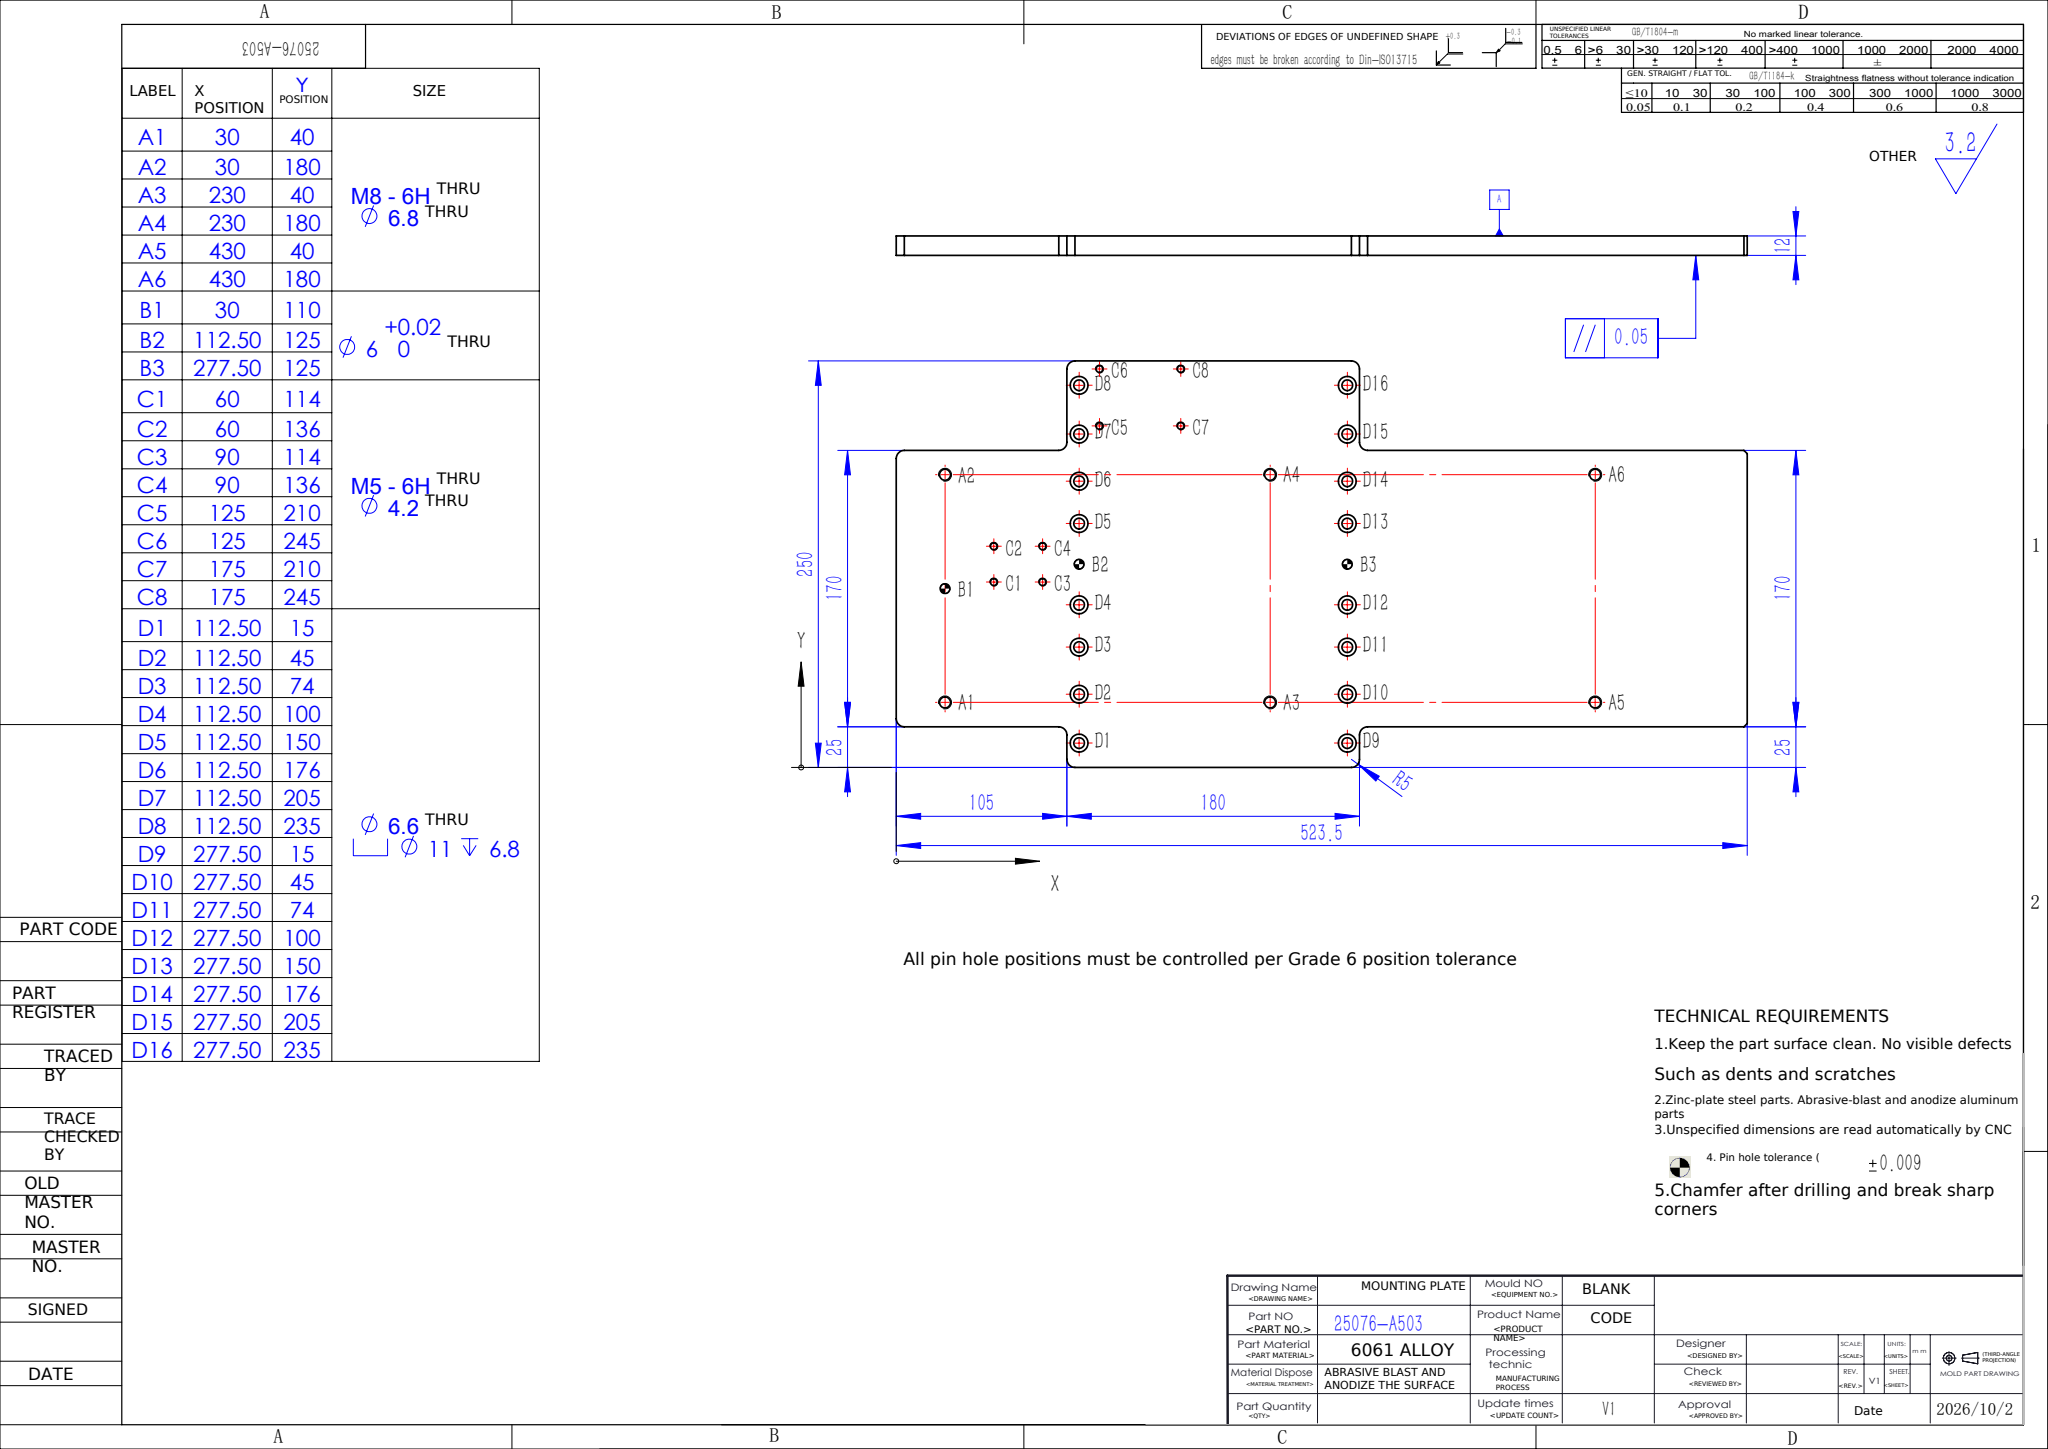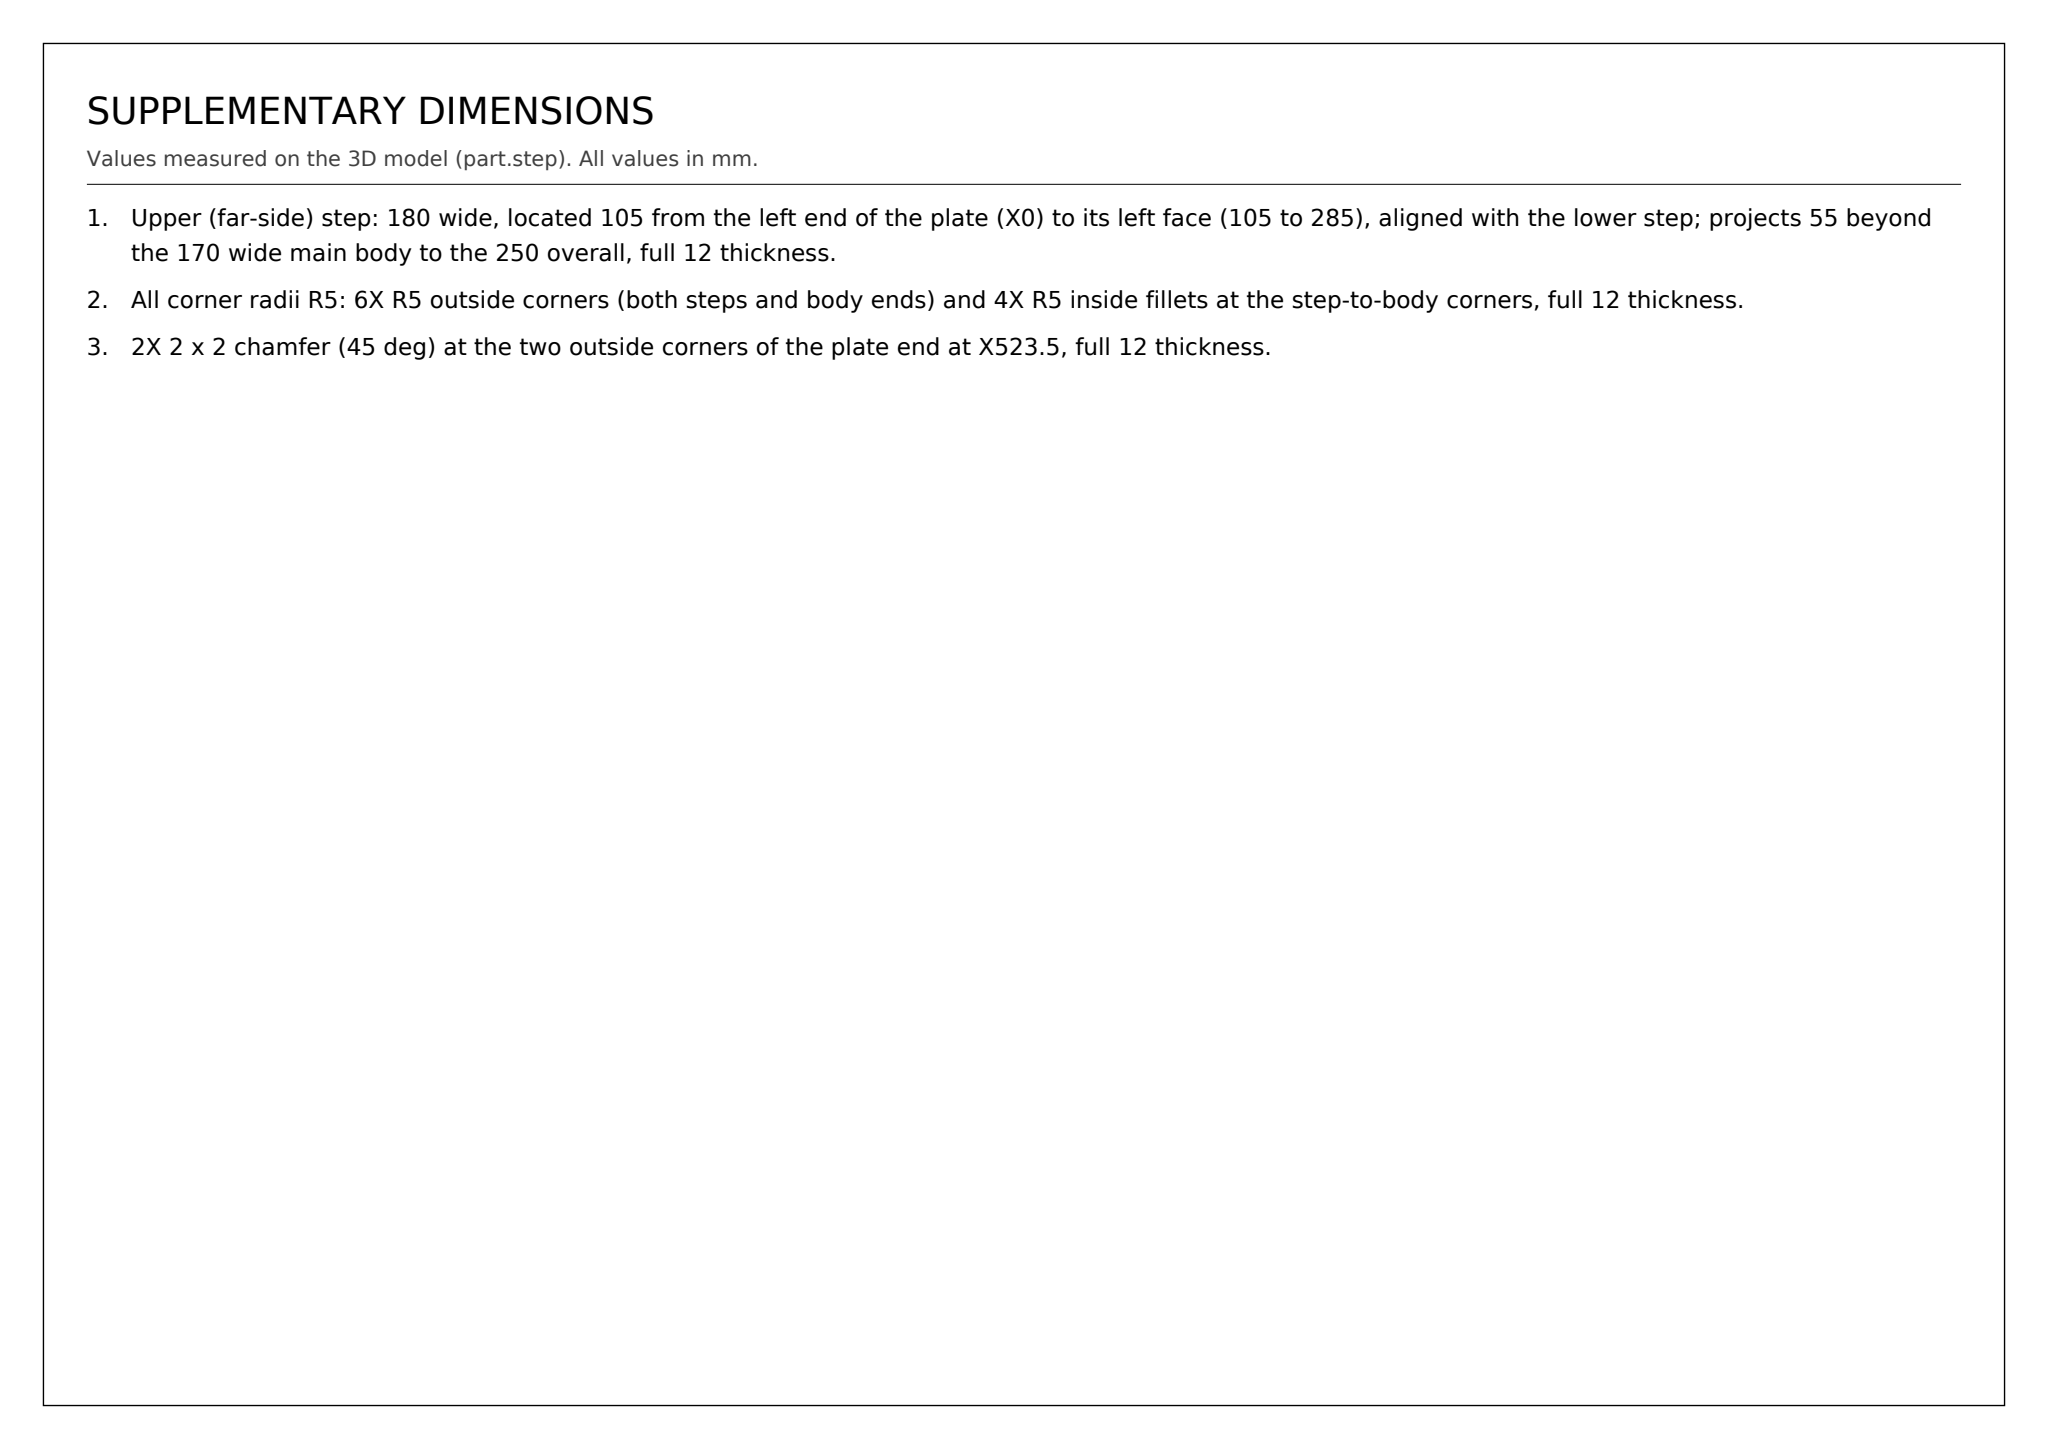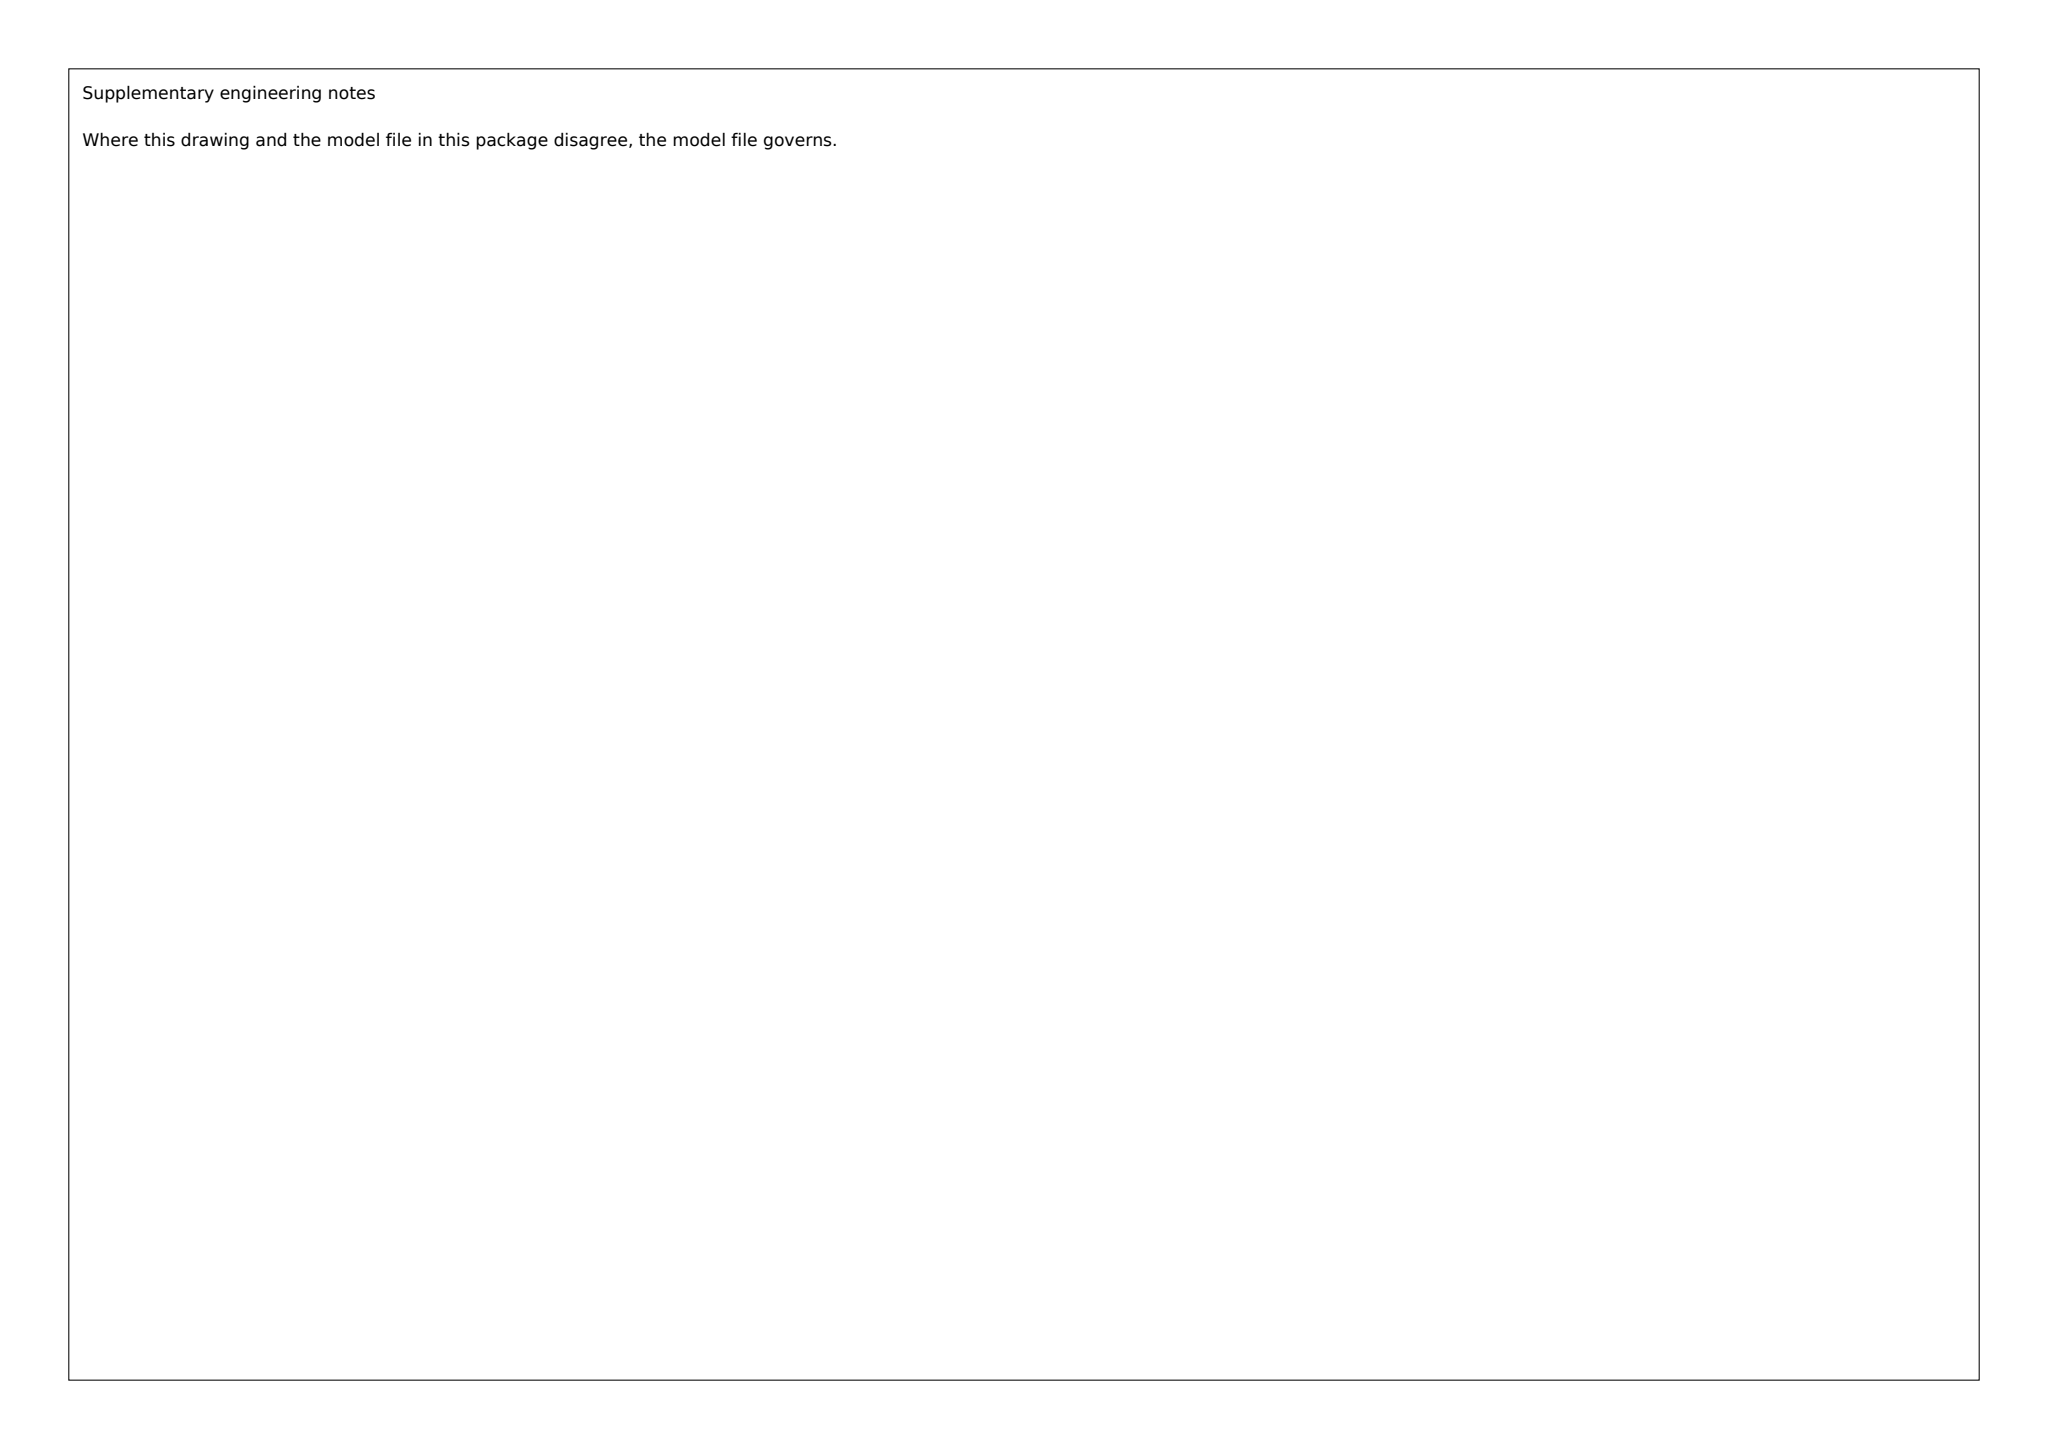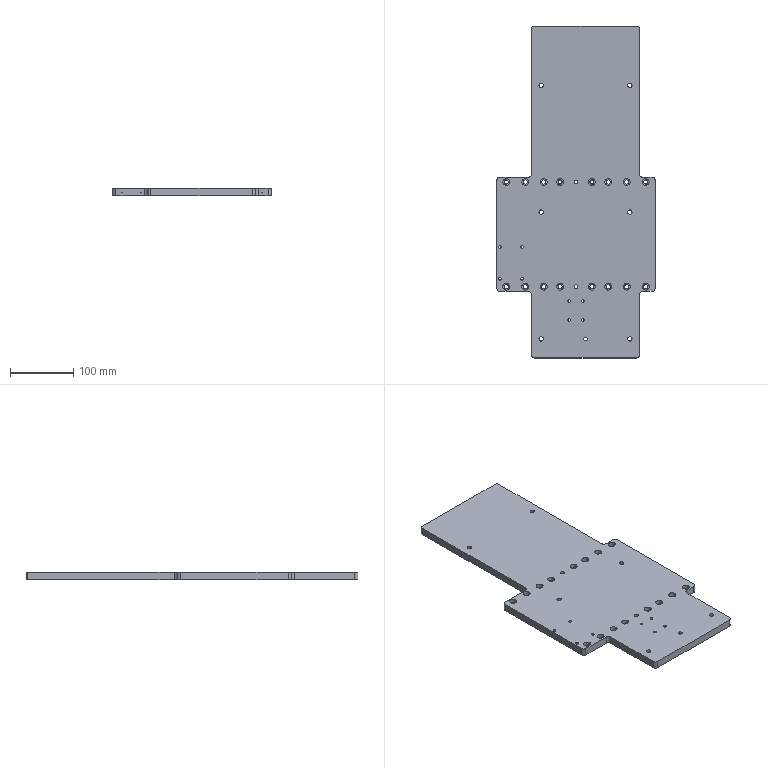Part | SolidWorks | mm | 1 solid | 140 faces | box 250 x 523.5 x 12 mm | volume 1222414 mm3 | cylinder 108 | plane 32 | commonest cylinder face diameters 11 x32 6.6 x32 4.2 x16 6.8 x12 10 x10 6 x6
Drawing notes:
Upper (far-side) step: 180 wide, located 105 from the left end of the plate (X0) to its left face (105 to 285), aligned with the lower step; projects 55 beyond the 170 wide main body to the 250 overall, full 12 thickness. | from the solid: Narrow main body faces at x=55 and x=225 (170 wide) run the full length; the wide section spans x=0 to 250 only between y=105 and y=285 (180 long, i.e. 105 from the y=0 end). Projections are therefore 55 (x 0-55, drawing upper side, since drawing Y = 250 - STEP x per A2 at Y180 = STEP x70) and 25 (x 225-250, drawing lower side); all faces extend z 0 to 12.
All corner radii R5: 6X R5 outside corners (both steps and body ends) and 4X R5 inside fillets at the step-to-body corners, full 12 thickness. | from the solid: cylinders: 6 convex arcs Ø10 (R5) 90 deg z 0-12 at (220,5),(60,5),(245,110),(245,280),(5,110),(5,280) and 4 concave arcs Ø10 (R5) 90 deg z 0-12 at (230,100),(230,290),(50,100),(50,290)
2X 2 x 2 chamfer (45 deg) at the two outside corners of the plate end at X523.5, full 12 thickness. | from the solid: inclined_planes 45/45/90 at bbox_from (223,521.5,0) and (55,521.5,0), size 2 x 2 x 12
build123d program:
from build123d import *

# Parameters (mm, degrees)
SKETCH1_W                                           = 140
SKETCH1_H                                           = 630
BOSS_EXTRUDE1_DEPTH                                 = 12
BOSS_EXTRUDE3_DEPTH                                 = 12
FILLET2_R                                           = 5
FILLET3_R                                           = 5
FILLET1_R                                           = 5
HOLE_SIZE_ACCORDING_TO_TYPE_3_OF_HEXAGO_D           = 6.6
HOLE_SIZE_ACCORDING_TO_TYPE_3_OF_HEXAGO_CBORE_D     = 11
HOLE_SIZE_ACCORDING_TO_TYPE_3_OF_HEXAGO_CBORE_DEPTH = 6.8
SIZE_MM_DOWEL_PIN_HOLE2_D                           = 6
M5_TAPPED_HOLE2_D                                   = 4.2
M5_TAPPED_HOLE3_D                                   = 4.2
M8_TAPPED_HOLE1_D                                   = 6.8
SIZE_MM_DOWEL_PIN_HOLE3_D                           = 6
SKETCH36_W                                          = 355.296
SKETCH36_H                                          = 153.423
CUT_EXTRUDE2_DEPTH                                  = 340.108
CHAMFER1_SIZE                                       = 2


with BuildPart() as part:
    # Sketch1 → Boss-Extrude1 (new body)
    with BuildSketch(Plane.XY):
        Rectangle(SKETCH1_W, SKETCH1_H)
    extrude(amount=BOSS_EXTRUDE1_DEPTH)

    # Sketch8 → Boss-Extrude3 (add, through all)
    with BuildSketch(Plane.XY.offset(12)):
        Polygon((70, -315), (100, -315), (100, -210), (125, -210), (125, -30), (100, -30), (100, 315), (70, 315), (70, -30), (-125, -30), (-125, -210), (70, -210), align=None)
    extrude(amount=-BOSS_EXTRUDE3_DEPTH)

    # Fillet2
    fillet2_edges = [part.edges().sort_by_distance(p)[0] for p in [
        (100, -30, 6),
        (100, -210, 6),
        (-70, -210, 6),
        (-70, -30, 6),
    ]]
    fillet(fillet2_edges, radius=FILLET2_R)

    # Fillet3
    fillet3_edges = [part.edges().sort_by_distance(p)[0] for p in [
        (-125, -30, 6),
        (125, -30, 6),
        (125, -210, 6),
        (-125, -210, 6),
    ]]
    fillet(fillet3_edges, radius=FILLET3_R)

    # Fillet1
    fillet1_edges = [part.edges().sort_by_distance(p)[0] for p in [
        (100, -315, 6),
        (100, 315, 6),
        (-70, -315, 6),
        (-70, 315, 6),
    ]]
    fillet(fillet1_edges, radius=FILLET1_R)

    # Hole Size_ According to_Type 3 of Hexago (through all)
    with Locations(Plane.XY.offset(12)):
        with Locations((110, -202.5), (80, -202.5), (51, -202.5), (25, -202.5), (-25, -202.5), (-51, -202.5), (-80, -202.5), (-110, -202.5), (-110, -37.5), (-80, -37.5), (-51, -37.5), (-25, -37.5), (25, -37.5), (51, -37.5), (80, -37.5), (110, -37.5)):
            CounterBoreHole(HOLE_SIZE_ACCORDING_TO_TYPE_3_OF_HEXAGO_D / 2, HOLE_SIZE_ACCORDING_TO_TYPE_3_OF_HEXAGO_CBORE_D / 2, HOLE_SIZE_ACCORDING_TO_TYPE_3_OF_HEXAGO_CBORE_DEPTH)

    # Size mm Dowel Pin Hole2 (through all)
    with Locations(Plane.XY.offset(12)):
        with Locations((0, -202.5), (0, -37.5)):
            Hole(SIZE_MM_DOWEL_PIN_HOLE2_D / 2)

    # M5 Tapped Hole2 (through all)
    with Locations(Plane.XY.offset(12)):
        with Locations((-85, -190), (-120, -190), (-120, -140), (-85, -140)):
            Hole(M5_TAPPED_HOLE2_D / 2)

    # M5 Tapped Hole3 (through all)
    with Locations(Plane(origin=(0, 0, 0), x_dir=(-1, 0, 0), z_dir=(0, 0, -1))):
        with Locations((11, -255), (11, -225), (-11, -225), (-11, -255)):
            Hole(M5_TAPPED_HOLE3_D / 2)

    # M8 Tapped Hole1 (through all)
    with Locations(Plane(origin=(0, 0, 0), x_dir=(-1, 0, 0), z_dir=(0, 0, -1))):
        with Locations((55, -285), (-85, -285), (55, -85), (-85, -85), (55, 115), (-85, 115), (55, 265), (-85, 265)):
            Hole(M8_TAPPED_HOLE1_D / 2)

    # Size mm Dowel Pin Hole3 (through all)
    with Locations(Plane(origin=(0, 0, 0), x_dir=(-1, 0, 0), z_dir=(0, 0, -1))):
        with Locations((-15, -285), (-15, 265)):
            Hole(SIZE_MM_DOWEL_PIN_HOLE3_D / 2)

    # Sketch36 → Cut-Extrude2 (cut, through all)
    with BuildSketch(Plane(origin=(0, 0, 0), x_dir=(-1, 0, 0), z_dir=(0, 0, -1))):
        with Locations((-33.502, 285.212)):
            Rectangle(SKETCH36_W, SKETCH36_H)
    extrude(amount=-CUT_EXTRUDE2_DEPTH, mode=Mode.SUBTRACT)

    # Chamfer1
    chamfer1_edges = [part.edges().sort_by_distance(p)[0] for p in [
        (100, 208.5, 6),
        (-70, 208.5, 6),
    ]]
    chamfer(chamfer1_edges, length=CHAMFER1_SIZE)


solid = part.part